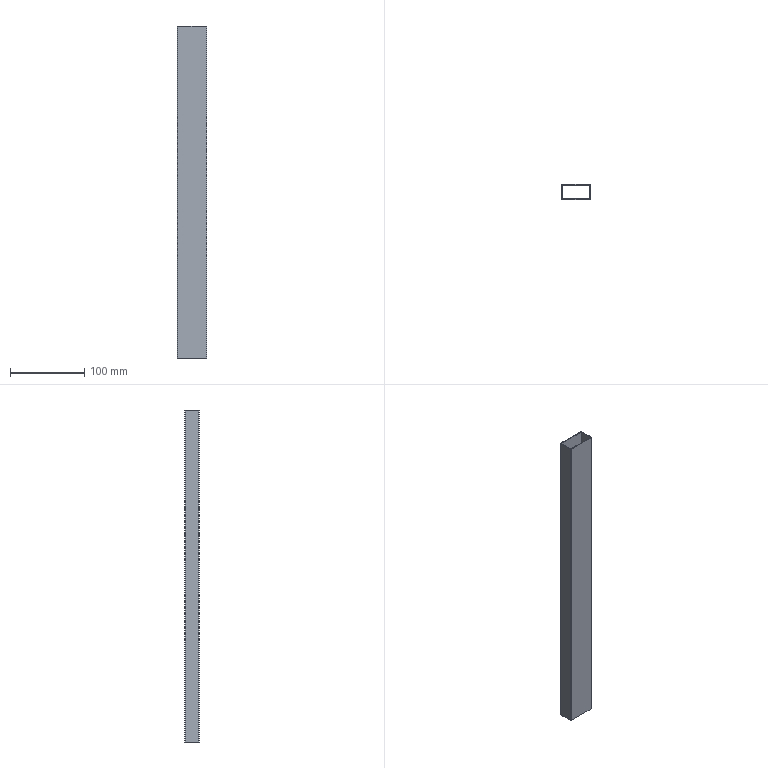Component | SolidWorks | DrawerStiffenerInner-1 | 1 solid | 14 faces | box 40 x 20 x 448.5 mm | volume 61616 mm3 | plane 10 | cylinder 4 | commonest cylinder face diameters 2 x4
build123d program:
from build123d import *

# Parameters (mm, degrees)
SKETCH1_W           = 17.6
SKETCH1_H           = 37.6
BOSS_EXTRUDE1_DEPTH = 448.5


with BuildPart() as part:
    # Sketch1 → Boss-Extrude1 (new body)
    with BuildSketch(Plane(origin=(0, 0, 0), x_dir=(1, 0, 0), z_dir=(0, 1, 0))):
        with BuildLine():
            Line((-9, 20), (9, 20))
            ThreePointArc((9, 20), (9.707, 19.707), (10, 19))
            Line((10, 19), (10, -19))
            ThreePointArc((10, -19), (9.707, -19.707), (9, -20))
            Line((9, -20), (-9, -20))
            ThreePointArc((-9, -20), (-9.707, -19.707), (-10, -19))
            Line((-10, -19), (-10, 19))
            ThreePointArc((-10, 19), (-9.707, 19.707), (-9, 20))
        make_face()
        Rectangle(SKETCH1_W, SKETCH1_H, mode=Mode.SUBTRACT)
    extrude(amount=BOSS_EXTRUDE1_DEPTH)


solid = part.part

# Placed as in the assembly
solid = solid.moved(Location((38.5, 246, -128.5), (90, -90, 0)))
STEP:
#1=COLOUR_RGB('',0.7922,0.8196,0.9333);
#2=FILL_AREA_STYLE_COLOUR('',#1);
#3=FILL_AREA_STYLE('',(#2));
#4=SURFACE_STYLE_FILL_AREA(#3);
#5=SURFACE_SIDE_STYLE('',(#4));
#6=SURFACE_STYLE_USAGE(.BOTH.,#5);
#7=PRESENTATION_STYLE_ASSIGNMENT((#6));
#8=CARTESIAN_POINT('',(0.7677,9.291,-5.059));
#9=VERTEX_POINT('',#8);
#10=CARTESIAN_POINT('',(0.7283,9.331,-5.059));
#11=VERTEX_POINT('',#10);
#12=CARTESIAN_POINT('',(0.7677,9.331,-5.059));
#13=DIRECTION('',(0.,-0.,-1.));
#14=DIRECTION('',(-1.,0.,0.));
#15=AXIS2_PLACEMENT_3D('',#12,#13,#14);
#16=CIRCLE('',#15,0.03937);
#17=EDGE_CURVE('',#9,#11,#16,.T.);
#18=ORIENTED_EDGE('',*,*,#17,.T.);
#19=CARTESIAN_POINT('',(0.7283,10.039,-5.059));
#20=VERTEX_POINT('',#19);
#21=CARTESIAN_POINT('',(0.7283,9.331,-5.059));
#22=DIRECTION('',(0.,1.,-0.));
#23=VECTOR('',#22,39.37);
#24=LINE('',#21,#23);
#25=EDGE_CURVE('',#11,#20,#24,.T.);
#26=ORIENTED_EDGE('',*,*,#25,.T.);
#27=CARTESIAN_POINT('',(0.7677,10.079,-5.059));
#28=VERTEX_POINT('',#27);
#29=CARTESIAN_POINT('',(0.7677,10.039,-5.059));
#30=DIRECTION('',(0.,-0.,-1.));
#31=DIRECTION('',(1.,0.,0.));
#32=AXIS2_PLACEMENT_3D('',#29,#30,#31);
#33=CIRCLE('',#32,0.03937);
#34=EDGE_CURVE('',#20,#28,#33,.T.);
#35=ORIENTED_EDGE('',*,*,#34,.T.);
#36=CARTESIAN_POINT('',(2.264,10.079,-5.059));
#37=VERTEX_POINT('',#36);
#38=CARTESIAN_POINT('',(2.264,10.079,-5.059));
#39=DIRECTION('',(1.,-0.,0.));
#40=VECTOR('',#39,39.37);
#41=LINE('',#38,#40);
#42=EDGE_CURVE('',#28,#37,#41,.T.);
#43=ORIENTED_EDGE('',*,*,#42,.T.);
#44=CARTESIAN_POINT('',(2.303,10.039,-5.059));
#45=VERTEX_POINT('',#44);
#46=CARTESIAN_POINT('',(2.264,10.039,-5.059));
#47=DIRECTION('',(0.,-0.,-1.));
#48=DIRECTION('',(-1.,0.,0.));
#49=AXIS2_PLACEMENT_3D('',#46,#47,#48);
#50=CIRCLE('',#49,0.03937);
#51=EDGE_CURVE('',#37,#45,#50,.T.);
#52=ORIENTED_EDGE('',*,*,#51,.T.);
#53=CARTESIAN_POINT('',(2.303,9.331,-5.059));
#54=VERTEX_POINT('',#53);
#55=CARTESIAN_POINT('',(2.303,9.331,-5.059));
#56=DIRECTION('',(-0.,-1.,0.));
#57=VECTOR('',#56,39.37);
#58=LINE('',#55,#57);
#59=EDGE_CURVE('',#45,#54,#58,.T.);
#60=ORIENTED_EDGE('',*,*,#59,.T.);
#61=CARTESIAN_POINT('',(2.264,9.291,-5.059));
#62=VERTEX_POINT('',#61);
#63=CARTESIAN_POINT('',(2.264,9.331,-5.059));
#64=DIRECTION('',(0.,-0.,-1.));
#65=DIRECTION('',(-1.,0.,0.));
#66=AXIS2_PLACEMENT_3D('',#63,#64,#65);
#67=CIRCLE('',#66,0.03937);
#68=EDGE_CURVE('',#54,#62,#67,.T.);
#69=ORIENTED_EDGE('',*,*,#68,.T.);
#70=CARTESIAN_POINT('',(2.264,9.291,-5.059));
#71=DIRECTION('',(-1.,0.,-0.));
#72=VECTOR('',#71,39.37);
#73=LINE('',#70,#72);
#74=EDGE_CURVE('',#62,#9,#73,.T.);
#75=ORIENTED_EDGE('',*,*,#74,.T.);
#76=EDGE_LOOP('',(#18,#26,#35,#43,#52,#60,#69,#75));
#77=FACE_OUTER_BOUND('',#76,.T.);
#78=CARTESIAN_POINT('',(2.256,9.339,-5.059));
#79=VERTEX_POINT('',#78);
#80=CARTESIAN_POINT('',(0.7756,9.339,-5.059));
#81=VERTEX_POINT('',#80);
#82=CARTESIAN_POINT('',(2.256,9.339,-5.059));
#83=DIRECTION('',(-1.,0.,-0.));
#84=VECTOR('',#83,39.37);
#85=LINE('',#82,#84);
#86=EDGE_CURVE('',#79,#81,#85,.T.);
#87=ORIENTED_EDGE('',*,*,#86,.F.);
#88=CARTESIAN_POINT('',(2.256,10.031,-5.059));
#89=VERTEX_POINT('',#88);
#90=CARTESIAN_POINT('',(2.256,9.339,-5.059));
#91=DIRECTION('',(-0.,-1.,0.));
#92=VECTOR('',#91,39.37);
#93=LINE('',#90,#92);
#94=EDGE_CURVE('',#89,#79,#93,.T.);
#95=ORIENTED_EDGE('',*,*,#94,.F.);
#96=CARTESIAN_POINT('',(0.7756,10.031,-5.059));
#97=VERTEX_POINT('',#96);
#98=CARTESIAN_POINT('',(2.256,10.031,-5.059));
#99=DIRECTION('',(1.,-0.,0.));
#100=VECTOR('',#99,39.37);
#101=LINE('',#98,#100);
#102=EDGE_CURVE('',#97,#89,#101,.T.);
#103=ORIENTED_EDGE('',*,*,#102,.F.);
#104=CARTESIAN_POINT('',(0.7756,9.339,-5.059));
#105=DIRECTION('',(0.,1.,-0.));
#106=VECTOR('',#105,39.37);
#107=LINE('',#104,#106);
#108=EDGE_CURVE('',#81,#97,#107,.T.);
#109=ORIENTED_EDGE('',*,*,#108,.F.);
#110=EDGE_LOOP('',(#87,#95,#103,#109));
#111=FACE_BOUND('',#110,.T.);
#112=CARTESIAN_POINT('',(0.7677,9.331,-5.059));
#113=DIRECTION('',(0.,-0.,-1.));
#114=DIRECTION('',(-1.,0.,-0.));
#115=AXIS2_PLACEMENT_3D('',#112,#113,#114);
#116=PLANE('',#115);
#117=ADVANCED_FACE('',(#77,#111),#116,.T.);
#118=CARTESIAN_POINT('',(0.7677,9.291,12.598));
#119=VERTEX_POINT('',#118);
#120=CARTESIAN_POINT('',(0.7283,9.331,12.598));
#121=VERTEX_POINT('',#120);
#122=CARTESIAN_POINT('',(0.7677,9.331,12.598));
#123=DIRECTION('',(0.,-0.,-1.));
#124=DIRECTION('',(-1.,0.,0.));
#125=AXIS2_PLACEMENT_3D('',#122,#123,#124);
#126=CIRCLE('',#125,0.03937);
#127=EDGE_CURVE('',#119,#121,#126,.T.);
#128=ORIENTED_EDGE('',*,*,#127,.F.);
#129=CARTESIAN_POINT('',(2.264,9.291,12.598));
#130=VERTEX_POINT('',#129);
#131=CARTESIAN_POINT('',(2.264,9.291,12.598));
#132=DIRECTION('',(-1.,0.,-0.));
#133=VECTOR('',#132,39.37);
#134=LINE('',#131,#133);
#135=EDGE_CURVE('',#130,#119,#134,.T.);
#136=ORIENTED_EDGE('',*,*,#135,.F.);
#137=CARTESIAN_POINT('',(2.303,9.331,12.598));
#138=VERTEX_POINT('',#137);
#139=CARTESIAN_POINT('',(2.264,9.331,12.598));
#140=DIRECTION('',(0.,-0.,-1.));
#141=DIRECTION('',(-1.,0.,0.));
#142=AXIS2_PLACEMENT_3D('',#139,#140,#141);
#143=CIRCLE('',#142,0.03937);
#144=EDGE_CURVE('',#138,#130,#143,.T.);
#145=ORIENTED_EDGE('',*,*,#144,.F.);
#146=CARTESIAN_POINT('',(2.303,10.039,12.598));
#147=VERTEX_POINT('',#146);
#148=CARTESIAN_POINT('',(2.303,9.331,12.598));
#149=DIRECTION('',(-0.,-1.,0.));
#150=VECTOR('',#149,39.37);
#151=LINE('',#148,#150);
#152=EDGE_CURVE('',#147,#138,#151,.T.);
#153=ORIENTED_EDGE('',*,*,#152,.F.);
#154=CARTESIAN_POINT('',(2.264,10.079,12.598));
#155=VERTEX_POINT('',#154);
#156=CARTESIAN_POINT('',(2.264,10.039,12.598));
#157=DIRECTION('',(0.,-0.,-1.));
#158=DIRECTION('',(-1.,0.,0.));
#159=AXIS2_PLACEMENT_3D('',#156,#157,#158);
#160=CIRCLE('',#159,0.03937);
#161=EDGE_CURVE('',#155,#147,#160,.T.);
#162=ORIENTED_EDGE('',*,*,#161,.F.);
#163=CARTESIAN_POINT('',(0.7677,10.079,12.598));
#164=VERTEX_POINT('',#163);
#165=CARTESIAN_POINT('',(2.264,10.079,12.598));
#166=DIRECTION('',(1.,-0.,0.));
#167=VECTOR('',#166,39.37);
#168=LINE('',#165,#167);
#169=EDGE_CURVE('',#164,#155,#168,.T.);
#170=ORIENTED_EDGE('',*,*,#169,.F.);
#171=CARTESIAN_POINT('',(0.7283,10.039,12.598));
#172=VERTEX_POINT('',#171);
#173=CARTESIAN_POINT('',(0.7677,10.039,12.598));
#174=DIRECTION('',(0.,-0.,-1.));
#175=DIRECTION('',(1.,0.,0.));
#176=AXIS2_PLACEMENT_3D('',#173,#174,#175);
#177=CIRCLE('',#176,0.03937);
#178=EDGE_CURVE('',#172,#164,#177,.T.);
#179=ORIENTED_EDGE('',*,*,#178,.F.);
#180=CARTESIAN_POINT('',(0.7283,9.331,12.598));
#181=DIRECTION('',(0.,1.,-0.));
#182=VECTOR('',#181,39.37);
#183=LINE('',#180,#182);
#184=EDGE_CURVE('',#121,#172,#183,.T.);
#185=ORIENTED_EDGE('',*,*,#184,.F.);
#186=EDGE_LOOP('',(#128,#136,#145,#153,#162,#170,#179,#185));
#187=FACE_OUTER_BOUND('',#186,.T.);
#188=CARTESIAN_POINT('',(2.256,10.031,12.598));
#189=VERTEX_POINT('',#188);
#190=CARTESIAN_POINT('',(2.256,9.339,12.598));
#191=VERTEX_POINT('',#190);
#192=CARTESIAN_POINT('',(2.256,9.339,12.598));
#193=DIRECTION('',(-0.,-1.,0.));
#194=VECTOR('',#193,39.37);
#195=LINE('',#192,#194);
#196=EDGE_CURVE('',#189,#191,#195,.T.);
#197=ORIENTED_EDGE('',*,*,#196,.T.);
#198=CARTESIAN_POINT('',(0.7756,9.339,12.598));
#199=VERTEX_POINT('',#198);
#200=CARTESIAN_POINT('',(2.256,9.339,12.598));
#201=DIRECTION('',(-1.,0.,-0.));
#202=VECTOR('',#201,39.37);
#203=LINE('',#200,#202);
#204=EDGE_CURVE('',#191,#199,#203,.T.);
#205=ORIENTED_EDGE('',*,*,#204,.T.);
#206=CARTESIAN_POINT('',(0.7756,10.031,12.598));
#207=VERTEX_POINT('',#206);
#208=CARTESIAN_POINT('',(0.7756,9.339,12.598));
#209=DIRECTION('',(0.,1.,-0.));
#210=VECTOR('',#209,39.37);
#211=LINE('',#208,#210);
#212=EDGE_CURVE('',#199,#207,#211,.T.);
#213=ORIENTED_EDGE('',*,*,#212,.T.);
#214=CARTESIAN_POINT('',(2.256,10.031,12.598));
#215=DIRECTION('',(1.,-0.,0.));
#216=VECTOR('',#215,39.37);
#217=LINE('',#214,#216);
#218=EDGE_CURVE('',#207,#189,#217,.T.);
#219=ORIENTED_EDGE('',*,*,#218,.T.);
#220=EDGE_LOOP('',(#197,#205,#213,#219));
#221=FACE_BOUND('',#220,.T.);
#222=CARTESIAN_POINT('',(0.7677,9.331,12.598));
#223=DIRECTION('',(0.,-0.,-1.));
#224=DIRECTION('',(-1.,0.,-0.));
#225=AXIS2_PLACEMENT_3D('',#222,#223,#224);
#226=PLANE('',#225);
#227=ADVANCED_FACE('',(#187,#221),#226,.F.);
#228=ORIENTED_EDGE('',*,*,#127,.T.);
#229=CARTESIAN_POINT('',(0.7283,9.331,-5.059));
#230=DIRECTION('',(-0.,0.,1.));
#231=VECTOR('',#230,39.37);
#232=LINE('',#229,#231);
#233=EDGE_CURVE('',#11,#121,#232,.T.);
#234=ORIENTED_EDGE('',*,*,#233,.F.);
#235=ORIENTED_EDGE('',*,*,#17,.F.);
#236=CARTESIAN_POINT('',(0.7677,9.291,-5.059));
#237=DIRECTION('',(-0.,0.,1.));
#238=VECTOR('',#237,39.37);
#239=LINE('',#236,#238);
#240=EDGE_CURVE('',#9,#119,#239,.T.);
#241=ORIENTED_EDGE('',*,*,#240,.T.);
#242=EDGE_LOOP('',(#228,#234,#235,#241));
#243=FACE_OUTER_BOUND('',#242,.T.);
#244=CARTESIAN_POINT('',(0.7677,9.331,-5.059));
#245=DIRECTION('',(-0.,0.,1.));
#246=DIRECTION('',(1.,0.,0.));
#247=AXIS2_PLACEMENT_3D('',#244,#245,#246);
#248=CYLINDRICAL_SURFACE('',#247,0.03937);
#249=ADVANCED_FACE('',(#243),#248,.T.);
#250=ORIENTED_EDGE('',*,*,#184,.T.);
#251=CARTESIAN_POINT('',(0.7283,10.039,-5.059));
#252=DIRECTION('',(-0.,0.,1.));
#253=VECTOR('',#252,39.37);
#254=LINE('',#251,#253);
#255=EDGE_CURVE('',#20,#172,#254,.T.);
#256=ORIENTED_EDGE('',*,*,#255,.F.);
#257=ORIENTED_EDGE('',*,*,#25,.F.);
#258=ORIENTED_EDGE('',*,*,#233,.T.);
#259=EDGE_LOOP('',(#250,#256,#257,#258));
#260=FACE_OUTER_BOUND('',#259,.T.);
#261=CARTESIAN_POINT('',(0.7283,9.331,-5.059));
#262=DIRECTION('',(1.,-0.,0.));
#263=DIRECTION('',(-0.,-1.,0.));
#264=AXIS2_PLACEMENT_3D('',#261,#262,#263);
#265=PLANE('',#264);
#266=ADVANCED_FACE('',(#260),#265,.F.);
#267=ORIENTED_EDGE('',*,*,#178,.T.);
#268=CARTESIAN_POINT('',(0.7677,10.079,-5.059));
#269=DIRECTION('',(-0.,0.,1.));
#270=VECTOR('',#269,39.37);
#271=LINE('',#268,#270);
#272=EDGE_CURVE('',#28,#164,#271,.T.);
#273=ORIENTED_EDGE('',*,*,#272,.F.);
#274=ORIENTED_EDGE('',*,*,#34,.F.);
#275=ORIENTED_EDGE('',*,*,#255,.T.);
#276=EDGE_LOOP('',(#267,#273,#274,#275));
#277=FACE_OUTER_BOUND('',#276,.T.);
#278=CARTESIAN_POINT('',(0.7677,10.039,-5.059));
#279=DIRECTION('',(-0.,0.,1.));
#280=DIRECTION('',(1.,0.,0.));
#281=AXIS2_PLACEMENT_3D('',#278,#279,#280);
#282=CYLINDRICAL_SURFACE('',#281,0.03937);
#283=ADVANCED_FACE('',(#277),#282,.T.);
#284=ORIENTED_EDGE('',*,*,#169,.T.);
#285=CARTESIAN_POINT('',(2.264,10.079,-5.059));
#286=DIRECTION('',(-0.,0.,1.));
#287=VECTOR('',#286,39.37);
#288=LINE('',#285,#287);
#289=EDGE_CURVE('',#37,#155,#288,.T.);
#290=ORIENTED_EDGE('',*,*,#289,.F.);
#291=ORIENTED_EDGE('',*,*,#42,.F.);
#292=ORIENTED_EDGE('',*,*,#272,.T.);
#293=EDGE_LOOP('',(#284,#290,#291,#292));
#294=FACE_OUTER_BOUND('',#293,.T.);
#295=CARTESIAN_POINT('',(2.264,10.079,-5.059));
#296=DIRECTION('',(-0.,-1.,0.));
#297=DIRECTION('',(-1.,0.,-0.));
#298=AXIS2_PLACEMENT_3D('',#295,#296,#297);
#299=PLANE('',#298);
#300=ADVANCED_FACE('',(#294),#299,.F.);
#301=ORIENTED_EDGE('',*,*,#161,.T.);
#302=CARTESIAN_POINT('',(2.303,10.039,-5.059));
#303=DIRECTION('',(-0.,0.,1.));
#304=VECTOR('',#303,39.37);
#305=LINE('',#302,#304);
#306=EDGE_CURVE('',#45,#147,#305,.T.);
#307=ORIENTED_EDGE('',*,*,#306,.F.);
#308=ORIENTED_EDGE('',*,*,#51,.F.);
#309=ORIENTED_EDGE('',*,*,#289,.T.);
#310=EDGE_LOOP('',(#301,#307,#308,#309));
#311=FACE_OUTER_BOUND('',#310,.T.);
#312=CARTESIAN_POINT('',(2.264,10.039,-5.059));
#313=DIRECTION('',(-0.,0.,1.));
#314=DIRECTION('',(1.,0.,0.));
#315=AXIS2_PLACEMENT_3D('',#312,#313,#314);
#316=CYLINDRICAL_SURFACE('',#315,0.03937);
#317=ADVANCED_FACE('',(#311),#316,.T.);
#318=ORIENTED_EDGE('',*,*,#152,.T.);
#319=CARTESIAN_POINT('',(2.303,9.331,-5.059));
#320=DIRECTION('',(-0.,0.,1.));
#321=VECTOR('',#320,39.37);
#322=LINE('',#319,#321);
#323=EDGE_CURVE('',#54,#138,#322,.T.);
#324=ORIENTED_EDGE('',*,*,#323,.F.);
#325=ORIENTED_EDGE('',*,*,#59,.F.);
#326=ORIENTED_EDGE('',*,*,#306,.T.);
#327=EDGE_LOOP('',(#318,#324,#325,#326));
#328=FACE_OUTER_BOUND('',#327,.T.);
#329=CARTESIAN_POINT('',(2.303,9.331,-5.059));
#330=DIRECTION('',(-1.,0.,-0.));
#331=DIRECTION('',(0.,1.,-0.));
#332=AXIS2_PLACEMENT_3D('',#329,#330,#331);
#333=PLANE('',#332);
#334=ADVANCED_FACE('',(#328),#333,.F.);
#335=ORIENTED_EDGE('',*,*,#144,.T.);
#336=CARTESIAN_POINT('',(2.264,9.291,-5.059));
#337=DIRECTION('',(-0.,0.,1.));
#338=VECTOR('',#337,39.37);
#339=LINE('',#336,#338);
#340=EDGE_CURVE('',#62,#130,#339,.T.);
#341=ORIENTED_EDGE('',*,*,#340,.F.);
#342=ORIENTED_EDGE('',*,*,#68,.F.);
#343=ORIENTED_EDGE('',*,*,#323,.T.);
#344=EDGE_LOOP('',(#335,#341,#342,#343));
#345=FACE_OUTER_BOUND('',#344,.T.);
#346=CARTESIAN_POINT('',(2.264,9.331,-5.059));
#347=DIRECTION('',(-0.,0.,1.));
#348=DIRECTION('',(1.,0.,0.));
#349=AXIS2_PLACEMENT_3D('',#346,#347,#348);
#350=CYLINDRICAL_SURFACE('',#349,0.03937);
#351=ADVANCED_FACE('',(#345),#350,.T.);
#352=ORIENTED_EDGE('',*,*,#135,.T.);
#353=ORIENTED_EDGE('',*,*,#240,.F.);
#354=ORIENTED_EDGE('',*,*,#74,.F.);
#355=ORIENTED_EDGE('',*,*,#340,.T.);
#356=EDGE_LOOP('',(#352,#353,#354,#355));
#357=FACE_OUTER_BOUND('',#356,.T.);
#358=CARTESIAN_POINT('',(2.264,9.291,-5.059));
#359=DIRECTION('',(0.,1.,-0.));
#360=DIRECTION('',(1.,-0.,0.));
#361=AXIS2_PLACEMENT_3D('',#358,#359,#360);
#362=PLANE('',#361);
#363=ADVANCED_FACE('',(#357),#362,.F.);
#364=ORIENTED_EDGE('',*,*,#196,.F.);
#365=CARTESIAN_POINT('',(2.256,10.031,-5.059));
#366=DIRECTION('',(-0.,0.,1.));
#367=VECTOR('',#366,39.37);
#368=LINE('',#365,#367);
#369=EDGE_CURVE('',#89,#189,#368,.T.);
#370=ORIENTED_EDGE('',*,*,#369,.F.);
#371=ORIENTED_EDGE('',*,*,#94,.T.);
#372=CARTESIAN_POINT('',(2.256,9.339,-5.059));
#373=DIRECTION('',(-0.,0.,1.));
#374=VECTOR('',#373,39.37);
#375=LINE('',#372,#374);
#376=EDGE_CURVE('',#79,#191,#375,.T.);
#377=ORIENTED_EDGE('',*,*,#376,.T.);
#378=EDGE_LOOP('',(#364,#370,#371,#377));
#379=FACE_OUTER_BOUND('',#378,.T.);
#380=CARTESIAN_POINT('',(2.256,9.339,-5.059));
#381=DIRECTION('',(-1.,0.,-0.));
#382=DIRECTION('',(0.,1.,-0.));
#383=AXIS2_PLACEMENT_3D('',#380,#381,#382);
#384=PLANE('',#383);
#385=ADVANCED_FACE('',(#379),#384,.T.);
#386=ORIENTED_EDGE('',*,*,#204,.F.);
#387=ORIENTED_EDGE('',*,*,#376,.F.);
#388=ORIENTED_EDGE('',*,*,#86,.T.);
#389=CARTESIAN_POINT('',(0.7756,9.339,-5.059));
#390=DIRECTION('',(-0.,0.,1.));
#391=VECTOR('',#390,39.37);
#392=LINE('',#389,#391);
#393=EDGE_CURVE('',#81,#199,#392,.T.);
#394=ORIENTED_EDGE('',*,*,#393,.T.);
#395=EDGE_LOOP('',(#386,#387,#388,#394));
#396=FACE_OUTER_BOUND('',#395,.T.);
#397=CARTESIAN_POINT('',(2.256,9.339,-5.059));
#398=DIRECTION('',(0.,1.,-0.));
#399=DIRECTION('',(1.,-0.,0.));
#400=AXIS2_PLACEMENT_3D('',#397,#398,#399);
#401=PLANE('',#400);
#402=ADVANCED_FACE('',(#396),#401,.T.);
#403=ORIENTED_EDGE('',*,*,#212,.F.);
#404=ORIENTED_EDGE('',*,*,#393,.F.);
#405=ORIENTED_EDGE('',*,*,#108,.T.);
#406=CARTESIAN_POINT('',(0.7756,10.031,-5.059));
#407=DIRECTION('',(-0.,0.,1.));
#408=VECTOR('',#407,39.37);
#409=LINE('',#406,#408);
#410=EDGE_CURVE('',#97,#207,#409,.T.);
#411=ORIENTED_EDGE('',*,*,#410,.T.);
#412=EDGE_LOOP('',(#403,#404,#405,#411));
#413=FACE_OUTER_BOUND('',#412,.T.);
#414=CARTESIAN_POINT('',(0.7756,9.339,-5.059));
#415=DIRECTION('',(1.,-0.,0.));
#416=DIRECTION('',(-0.,-1.,0.));
#417=AXIS2_PLACEMENT_3D('',#414,#415,#416);
#418=PLANE('',#417);
#419=ADVANCED_FACE('',(#413),#418,.T.);
#420=ORIENTED_EDGE('',*,*,#218,.F.);
#421=ORIENTED_EDGE('',*,*,#410,.F.);
#422=ORIENTED_EDGE('',*,*,#102,.T.);
#423=ORIENTED_EDGE('',*,*,#369,.T.);
#424=EDGE_LOOP('',(#420,#421,#422,#423));
#425=FACE_OUTER_BOUND('',#424,.T.);
#426=CARTESIAN_POINT('',(2.256,10.031,-5.059));
#427=DIRECTION('',(-0.,-1.,0.));
#428=DIRECTION('',(-1.,0.,-0.));
#429=AXIS2_PLACEMENT_3D('',#426,#427,#428);
#430=PLANE('',#429);
#431=ADVANCED_FACE('',(#425),#430,.T.);
#432=CLOSED_SHELL('',(#117,#227,#249,#266,#283,#300,#317,#334,#351,#363,#385,#402,#419,#431));
#433=MANIFOLD_SOLID_BREP('',#432);
#434=STYLED_ITEM('',(#7),#433);
#435=PRESENTATION_LAYER_ASSIGNMENT('','',(#434));
#436=CARTESIAN_POINT('',(0.,0.,0.));
#437=DIRECTION('',(0.,0.,1.));
#438=DIRECTION('',(1.,0.,0.));
#439=AXIS2_PLACEMENT_3D('',#436,#437,#438);
#440=(LENGTH_UNIT()NAMED_UNIT(*)SI_UNIT($,.METRE.));
#441=LENGTH_MEASURE_WITH_UNIT(LENGTH_MEASURE(0.0254),#440);
#442=DIMENSIONAL_EXPONENTS(1.,0.,0.,0.,0.,0.,0.);
#443=(CONVERSION_BASED_UNIT('',#441)LENGTH_UNIT()NAMED_UNIT(#442));
#444=UNCERTAINTY_MEASURE_WITH_UNIT(LENGTH_MEASURE(0.00001),#443,'','');
#445=(NAMED_UNIT(*)PLANE_ANGLE_UNIT()SI_UNIT($,.RADIAN.));
#446=(NAMED_UNIT(*)SI_UNIT($,.STERADIAN.)SOLID_ANGLE_UNIT());
#447=(GEOMETRIC_REPRESENTATION_CONTEXT(3)GLOBAL_UNCERTAINTY_ASSIGNED_CONTEXT((#444))GLOBAL_UNIT_ASSIGNED_CONTEXT((#443,#445,#446))REPRESENTATION_CONTEXT('',''));
#448=ADVANCED_BREP_SHAPE_REPRESENTATION('',(#433,#439),#447);
#449=(LENGTH_UNIT()NAMED_UNIT(*)SI_UNIT($,.METRE.));
#450=LENGTH_MEASURE_WITH_UNIT(LENGTH_MEASURE(0.0254),#449);
#451=DIMENSIONAL_EXPONENTS(1.,0.,0.,0.,0.,0.,0.);
#452=(CONVERSION_BASED_UNIT('',#450)LENGTH_UNIT()NAMED_UNIT(#451));
#453=UNCERTAINTY_MEASURE_WITH_UNIT(LENGTH_MEASURE(0.00001),#452,'','');
#454=(NAMED_UNIT(*)PLANE_ANGLE_UNIT()SI_UNIT($,.RADIAN.));
#455=(NAMED_UNIT(*)SI_UNIT($,.STERADIAN.)SOLID_ANGLE_UNIT());
#456=(GEOMETRIC_REPRESENTATION_CONTEXT(3)GLOBAL_UNCERTAINTY_ASSIGNED_CONTEXT((#453))GLOBAL_UNIT_ASSIGNED_CONTEXT((#452,#454,#455))REPRESENTATION_CONTEXT('',''));
#457=MECHANICAL_DESIGN_GEOMETRIC_PRESENTATION_REPRESENTATION('',(#434),#456);